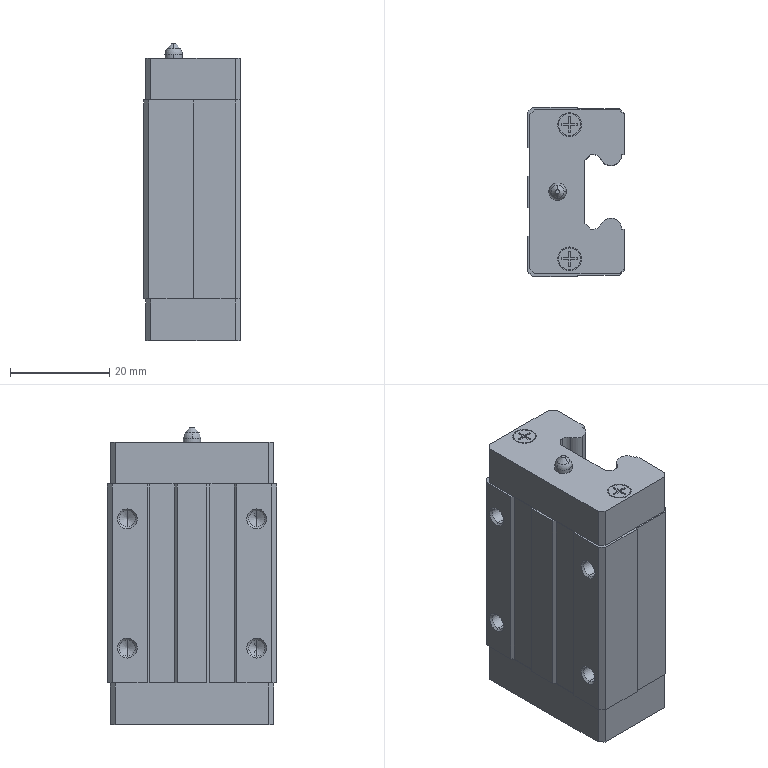Component | SolidWorks | SXRZ24_280-2_block_SXRB24-2 | 1 solid | 170 faces | box 19.4 x 34 x 59.8 mm | volume 30273 mm3 | plane 99 | cylinder 51 | cone 18 | sphere 2 | commonest cylinder face diameters 3.08 x20 4.4 x11 3.242 x8 4.8 x8 3.5 x2 3 x2
build123d program:
from build123d import *

# Parameters (mm, degrees)
BOSS_EXTRUDE1_DEPTH      = 20
BOSS_EXTRUDE1_DEPTH_BACK = 20
BOSS_EXTRUDE2_DEPTH      = 8.4
BOSS_EXTRUDE3_START      = -8.4
BOSS_EXTRUDE3_DEPTH      = 8.4
SKETCH5_R                = 2.4
CUT_EXTRUDE1_DEPTH       = 2.5
SKETCH6_R                = 2.4
CUT_EXTRUDE2_DEPTH       = 2.5
CUT_EXTRUDE3_START       = -2.5
SKETCH7_R                = 2.4
CUT_EXTRUDE3_DEPTH       = 2.5
CUT_EXTRUDE4_START       = -2.5
SKETCH8_R                = 2.4
CUT_EXTRUDE4_DEPTH       = 2.5
SKETCH9_R                = 2.2
BOSS_EXTRUDE4_DEPTH      = 2.5
SKETCH10_R               = 2.2
BOSS_EXTRUDE5_DEPTH      = 2.5
BOSS_EXTRUDE6_START      = 2.5
SKETCH11_R               = 2.2
BOSS_EXTRUDE6_DEPTH      = 2.5
BOSS_EXTRUDE7_START      = 2.5
SKETCH12_R               = 2.2
BOSS_EXTRUDE7_DEPTH      = 2.5
CUT_EXTRUDE5_DEPTH       = 0.2
CUT_EXTRUDE6_DEPTH       = 0.2
CUT_EXTRUDE7_START       = 0.2
CUT_EXTRUDE7_DEPTH       = 0.2
CUT_EXTRUDE8_START       = 0.2
CUT_EXTRUDE8_DEPTH       = 0.2
LPATTERN1_COUNT          = 2
LPATTERN1_PITCH          = 26
LPATTERN1_COUNT_DIR2     = 2
LPATTERN1_PITCH_DIR2     = 26


with BuildPart() as part:
    # Sketch1 → Boss-Extrude1 (new, two sides: drawn at the far end of the back side and taken through both)
    with BuildSketch(Plane.XY.offset(-BOSS_EXTRUDE1_DEPTH_BACK)):
        with BuildLine():
            Line((-17, 18.41), (-17, 9.4))
            Line((-17, 9.4), (-16.75, 9.4))
            Line((-16.75, 9.4), (-16.75, 0.997))
            Line((-16.75, 0.997), (-15.753, 0))
            Line((-15.753, 0), (-7.5, 0))
            Line((-7.5, 0), (-7.5, 0.505))
            ThreePointArc((-7.5, 0.505), (-5.348, 2.249), (-6.608, 4.716))
            ThreePointArc((-6.608, 4.716), (-7.257, 5.269), (-7.5, 6.087))
            Line((-7.5, 6.087), (-7.5, 6.776))
            Line((-7.5, 6.776), (-6.376, 7.9))
            Line((-6.376, 7.9), (6.376, 7.9))
            Line((6.376, 7.9), (7.5, 6.776))
            Line((7.5, 6.776), (7.5, 6.087))
            ThreePointArc((7.5, 6.087), (7.257, 5.269), (6.608, 4.716))
            ThreePointArc((6.608, 4.716), (5.348, 2.249), (7.5, 0.505))
            Line((7.5, 0.505), (7.5, 0))
            Line((7.5, 0), (15.753, 0))
            Line((15.753, 0), (16.75, 0.997))
            Line((16.75, 0.997), (16.75, 9.4))
            Line((16.75, 9.4), (17, 9.4))
            Line((17, 9.4), (17, 18.41))
            Line((17, 18.41), (16.01, 19.4))
            Line((16.01, 19.4), (9, 19.4))
            Line((9, 19.4), (8.5, 18.9))
            Line((8.5, 18.9), (3.5, 18.9))
            Line((3.5, 18.9), (3, 19.4))
            Line((3, 19.4), (-3, 19.4))
            Line((-3, 19.4), (-3.5, 18.9))
            Line((-3.5, 18.9), (-8.5, 18.9))
            Line((-8.5, 18.9), (-9, 19.4))
            Line((-9, 19.4), (-16.01, 19.4))
            Line((-16.01, 19.4), (-17, 18.41))
        make_face()
    extrude(amount=BOSS_EXTRUDE1_DEPTH + BOSS_EXTRUDE1_DEPTH_BACK)

    # Sketch2 → Boss-Extrude2 (add)
    with BuildSketch(Plane.XY.offset(20)):
        with BuildLine():
            Line((-16.45, 18.01), (-16.45, 0.997))
            Line((-16.45, 0.997), (-15.453, 0))
            Line((-15.453, 0), (-7.5, 0))
            Line((-7.5, 0), (-7.5, 0.505))
            ThreePointArc((-7.5, 0.505), (-5.348, 2.249), (-6.608, 4.716))
            ThreePointArc((-6.608, 4.716), (-7.257, 5.269), (-7.5, 6.087))
            Line((-7.5, 6.087), (-7.5, 6.776))
            Line((-7.5, 6.776), (-6.376, 7.9))
            Line((-6.376, 7.9), (6.376, 7.9))
            Line((6.376, 7.9), (7.5, 6.776))
            Line((7.5, 6.776), (7.5, 6.087))
            ThreePointArc((7.5, 6.087), (7.257, 5.269), (6.608, 4.716))
            ThreePointArc((6.608, 4.716), (5.348, 2.249), (7.5, 0.505))
            Line((7.5, 0.505), (7.5, 0))
            Line((7.5, 0), (15.453, 0))
            Line((15.453, 0), (16.45, 0.997))
            Line((16.45, 0.997), (16.45, 18.01))
            Line((16.45, 18.01), (15.46, 19))
            Line((15.46, 19), (-15.46, 19))
            Line((-15.46, 19), (-16.45, 18.01))
        make_face()
    extrude(amount=BOSS_EXTRUDE2_DEPTH)

    # Sketch3 → Boss-Extrude3 (add)
    with BuildSketch(Plane.XY.offset(-20).offset(BOSS_EXTRUDE3_START)):
        with BuildLine():
            Line((-16.45, 18.01), (-16.45, 0.997))
            Line((-16.45, 0.997), (-15.453, 0))
            Line((-15.453, 0), (-7.5, 0))
            Line((-7.5, 0), (-7.5, 0.505))
            ThreePointArc((-7.5, 0.505), (-5.348, 2.249), (-6.608, 4.716))
            ThreePointArc((-6.608, 4.716), (-7.257, 5.269), (-7.5, 6.087))
            Line((-7.5, 6.087), (-7.5, 6.776))
            Line((-7.5, 6.776), (-6.376, 7.9))
            Line((-6.376, 7.9), (6.376, 7.9))
            Line((6.376, 7.9), (7.5, 6.776))
            Line((7.5, 6.776), (7.5, 6.087))
            ThreePointArc((7.5, 6.087), (7.257, 5.269), (6.608, 4.716))
            ThreePointArc((6.608, 4.716), (5.348, 2.249), (7.5, 0.505))
            Line((7.5, 0.505), (7.5, 0))
            Line((7.5, 0), (15.453, 0))
            Line((15.453, 0), (16.45, 0.997))
            Line((16.45, 0.997), (16.45, 18.01))
            Line((16.45, 18.01), (15.46, 19))
            Line((15.46, 19), (-15.46, 19))
            Line((-15.46, 19), (-16.45, 18.01))
        make_face()
    extrude(amount=BOSS_EXTRUDE3_DEPTH)

    # Sketch4 → Cut-Revolve1 (revolve, cut)
    with BuildSketch(Plane(origin=(13, 0, 0), x_dir=(0, 0, -1), z_dir=(1, 0, 0)), mode=Mode.PRIVATE) as cut_revolve1_sk:
        Polygon((13, 19.4), (15, 19.4), (14.621, 19.021), (14.621, 10.336), (13, 9.4), align=None)
    cut_revolve1 = revolve(cut_revolve1_sk.sketch.rotate(Axis((13, 9.4, -13), (0, 1, 0)), 180), axis=Axis((13, 9.4, -13), (0, 1, 0)), mode=Mode.SUBTRACT)

    # Sketch5 → Cut-Extrude1 (cut)
    with BuildSketch(Plane.XY.offset(-28.4)):
        with Locations((-13.5, 11)):
            Circle(SKETCH5_R)
    extrude(amount=CUT_EXTRUDE1_DEPTH, mode=Mode.SUBTRACT)

    # Sketch6 → Cut-Extrude2 (cut)
    with BuildSketch(Plane.XY.offset(-28.4)):
        with Locations((13.5, 11)):
            Circle(SKETCH6_R)
    extrude(amount=CUT_EXTRUDE2_DEPTH, mode=Mode.SUBTRACT)

    # Sketch7 → Cut-Extrude3 (cut)
    with BuildSketch(Plane.XY.offset(28.4).offset(CUT_EXTRUDE3_START)):
        with Locations((-13.5, 11)):
            Circle(SKETCH7_R)
    extrude(amount=CUT_EXTRUDE3_DEPTH, mode=Mode.SUBTRACT)

    # Sketch8 → Cut-Extrude4 (cut)
    with BuildSketch(Plane.XY.offset(28.4).offset(CUT_EXTRUDE4_START)):
        with Locations((13.5, 11)):
            Circle(SKETCH8_R)
    extrude(amount=CUT_EXTRUDE4_DEPTH, mode=Mode.SUBTRACT)

    # Sketch9 → Boss-Extrude4 (add)
    with BuildSketch(Plane.XY.offset(28.4)):
        with Locations((-13.5, 11)):
            Circle(SKETCH9_R)
    extrude(amount=-BOSS_EXTRUDE4_DEPTH)

    # Sketch10 → Boss-Extrude5 (add)
    with BuildSketch(Plane.XY.offset(28.4)):
        with Locations((13.5, 11)):
            Circle(SKETCH10_R)
    extrude(amount=-BOSS_EXTRUDE5_DEPTH)

    # Sketch11 → Boss-Extrude6 (add)
    with BuildSketch(Plane.XY.offset(-28.4).offset(BOSS_EXTRUDE6_START)):
        with Locations((-13.5, 11)):
            Circle(SKETCH11_R)
    extrude(amount=-BOSS_EXTRUDE6_DEPTH)

    # Sketch12 → Boss-Extrude7 (add)
    with BuildSketch(Plane.XY.offset(-28.4).offset(BOSS_EXTRUDE7_START)):
        with Locations((13.5, 11)):
            Circle(SKETCH12_R)
    extrude(amount=-BOSS_EXTRUDE7_DEPTH)

    # Sketch13 → Cut-Extrude5 (cut)
    with BuildSketch(Plane.XY.offset(28.4)):
        with BuildLine():
            Line((-15.027, 10.8), (-13.7, 10.8))
            Line((-13.7, 10.8), (-13.7, 9.473))
            ThreePointArc((-13.7, 9.473), (-13.5, 9.46), (-13.3, 9.473))
            Line((-13.3, 9.473), (-13.3, 10.8))
            Line((-13.3, 10.8), (-11.973, 10.8))
            ThreePointArc((-11.973, 10.8), (-11.96, 11), (-11.973, 11.2))
            Line((-11.973, 11.2), (-13.3, 11.2))
            Line((-13.3, 11.2), (-13.3, 12.527))
            ThreePointArc((-13.3, 12.527), (-13.5, 12.54), (-13.7, 12.527))
            Line((-13.7, 12.527), (-13.7, 11.2))
            Line((-13.7, 11.2), (-15.027, 11.2))
            ThreePointArc((-15.027, 11.2), (-15.04, 11), (-15.027, 10.8))
        make_face()
    extrude(amount=-CUT_EXTRUDE5_DEPTH, mode=Mode.SUBTRACT)

    # Sketch14 → Cut-Extrude6 (cut)
    with BuildSketch(Plane.XY.offset(28.4)):
        with BuildLine():
            Line((11.973, 10.8), (13.3, 10.8))
            Line((13.3, 10.8), (13.3, 9.473))
            ThreePointArc((13.3, 9.473), (13.5, 9.46), (13.7, 9.473))
            Line((13.7, 9.473), (13.7, 10.8))
            Line((13.7, 10.8), (15.027, 10.8))
            ThreePointArc((15.027, 10.8), (15.04, 11), (15.027, 11.2))
            Line((15.027, 11.2), (13.7, 11.2))
            Line((13.7, 11.2), (13.7, 12.527))
            ThreePointArc((13.7, 12.527), (13.5, 12.54), (13.3, 12.527))
            Line((13.3, 12.527), (13.3, 11.2))
            Line((13.3, 11.2), (11.973, 11.2))
            ThreePointArc((11.973, 11.2), (11.96, 11), (11.973, 10.8))
        make_face()
    extrude(amount=-CUT_EXTRUDE6_DEPTH, mode=Mode.SUBTRACT)

    # Sketch15 → Cut-Extrude7 (cut)
    with BuildSketch(Plane.XY.offset(-28.4).offset(CUT_EXTRUDE7_START)):
        with BuildLine():
            Line((-15.027, 10.8), (-13.7, 10.8))
            Line((-13.7, 10.8), (-13.7, 9.473))
            ThreePointArc((-13.7, 9.473), (-13.5, 9.46), (-13.3, 9.473))
            Line((-13.3, 9.473), (-13.3, 10.8))
            Line((-13.3, 10.8), (-11.973, 10.8))
            ThreePointArc((-11.973, 10.8), (-11.96, 11), (-11.973, 11.2))
            Line((-11.973, 11.2), (-13.3, 11.2))
            Line((-13.3, 11.2), (-13.3, 12.527))
            ThreePointArc((-13.3, 12.527), (-13.5, 12.54), (-13.7, 12.527))
            Line((-13.7, 12.527), (-13.7, 11.2))
            Line((-13.7, 11.2), (-15.027, 11.2))
            ThreePointArc((-15.027, 11.2), (-15.04, 11), (-15.027, 10.8))
        make_face()
    extrude(amount=-CUT_EXTRUDE7_DEPTH, mode=Mode.SUBTRACT)

    # Sketch16 → Cut-Extrude8 (cut)
    with BuildSketch(Plane.XY.offset(-28.4).offset(CUT_EXTRUDE8_START)):
        with BuildLine():
            Line((11.973, 10.8), (13.3, 10.8))
            Line((13.3, 10.8), (13.3, 9.473))
            ThreePointArc((13.3, 9.473), (13.5, 9.46), (13.7, 9.473))
            Line((13.7, 9.473), (13.7, 10.8))
            Line((13.7, 10.8), (15.027, 10.8))
            ThreePointArc((15.027, 10.8), (15.04, 11), (15.027, 11.2))
            Line((15.027, 11.2), (13.7, 11.2))
            Line((13.7, 11.2), (13.7, 12.527))
            ThreePointArc((13.7, 12.527), (13.5, 12.54), (13.3, 12.527))
            Line((13.3, 12.527), (13.3, 11.2))
            Line((13.3, 11.2), (11.973, 11.2))
            ThreePointArc((11.973, 11.2), (11.96, 11), (11.973, 10.8))
        make_face()
    extrude(amount=-CUT_EXTRUDE8_DEPTH, mode=Mode.SUBTRACT)

    # Sketch17 → Revolve1 (revolve)
    with BuildSketch(Plane(origin=(0, 0, 0), x_dir=(0, 0, -1), z_dir=(1, 0, 0)), mode=Mode.PRIVATE) as revolve1_sk:
        with BuildLine():
            Line((-31.4, 13.4), (-31.4, 13.82))
            Line((-31.4, 13.82), (-30.387, 14.713))
            ThreePointArc((-30.387, 14.713), (-29.849, 15.037), (-29.23, 15.15))
            Line((-29.23, 15.15), (-28.4, 15.15))
            Line((-28.4, 15.15), (-28.4, 13.4))
            Line((-28.4, 13.4), (-31.4, 13.4))
        make_face()
    revolve(revolve1_sk.sketch.rotate(Axis((0, 13.4, 28.4), (0, 0, 1)), 90), axis=Axis((0, 13.4, 28.4), (0, 0, 1)))

    # LPattern1: Cut-Revolve1 2 × 2
    with Locations(*[(-i * LPATTERN1_PITCH, 0, j * LPATTERN1_PITCH_DIR2) for i in range(LPATTERN1_COUNT) for j in range(LPATTERN1_COUNT_DIR2) if (i, j) != (0, 0)]):
        add(cut_revolve1, mode=Mode.SUBTRACT)


solid = part.part

# Placed as in the assembly
solid = solid.moved(Location((-776.735, 517.593, 1071.877), (0, 0, 90)))